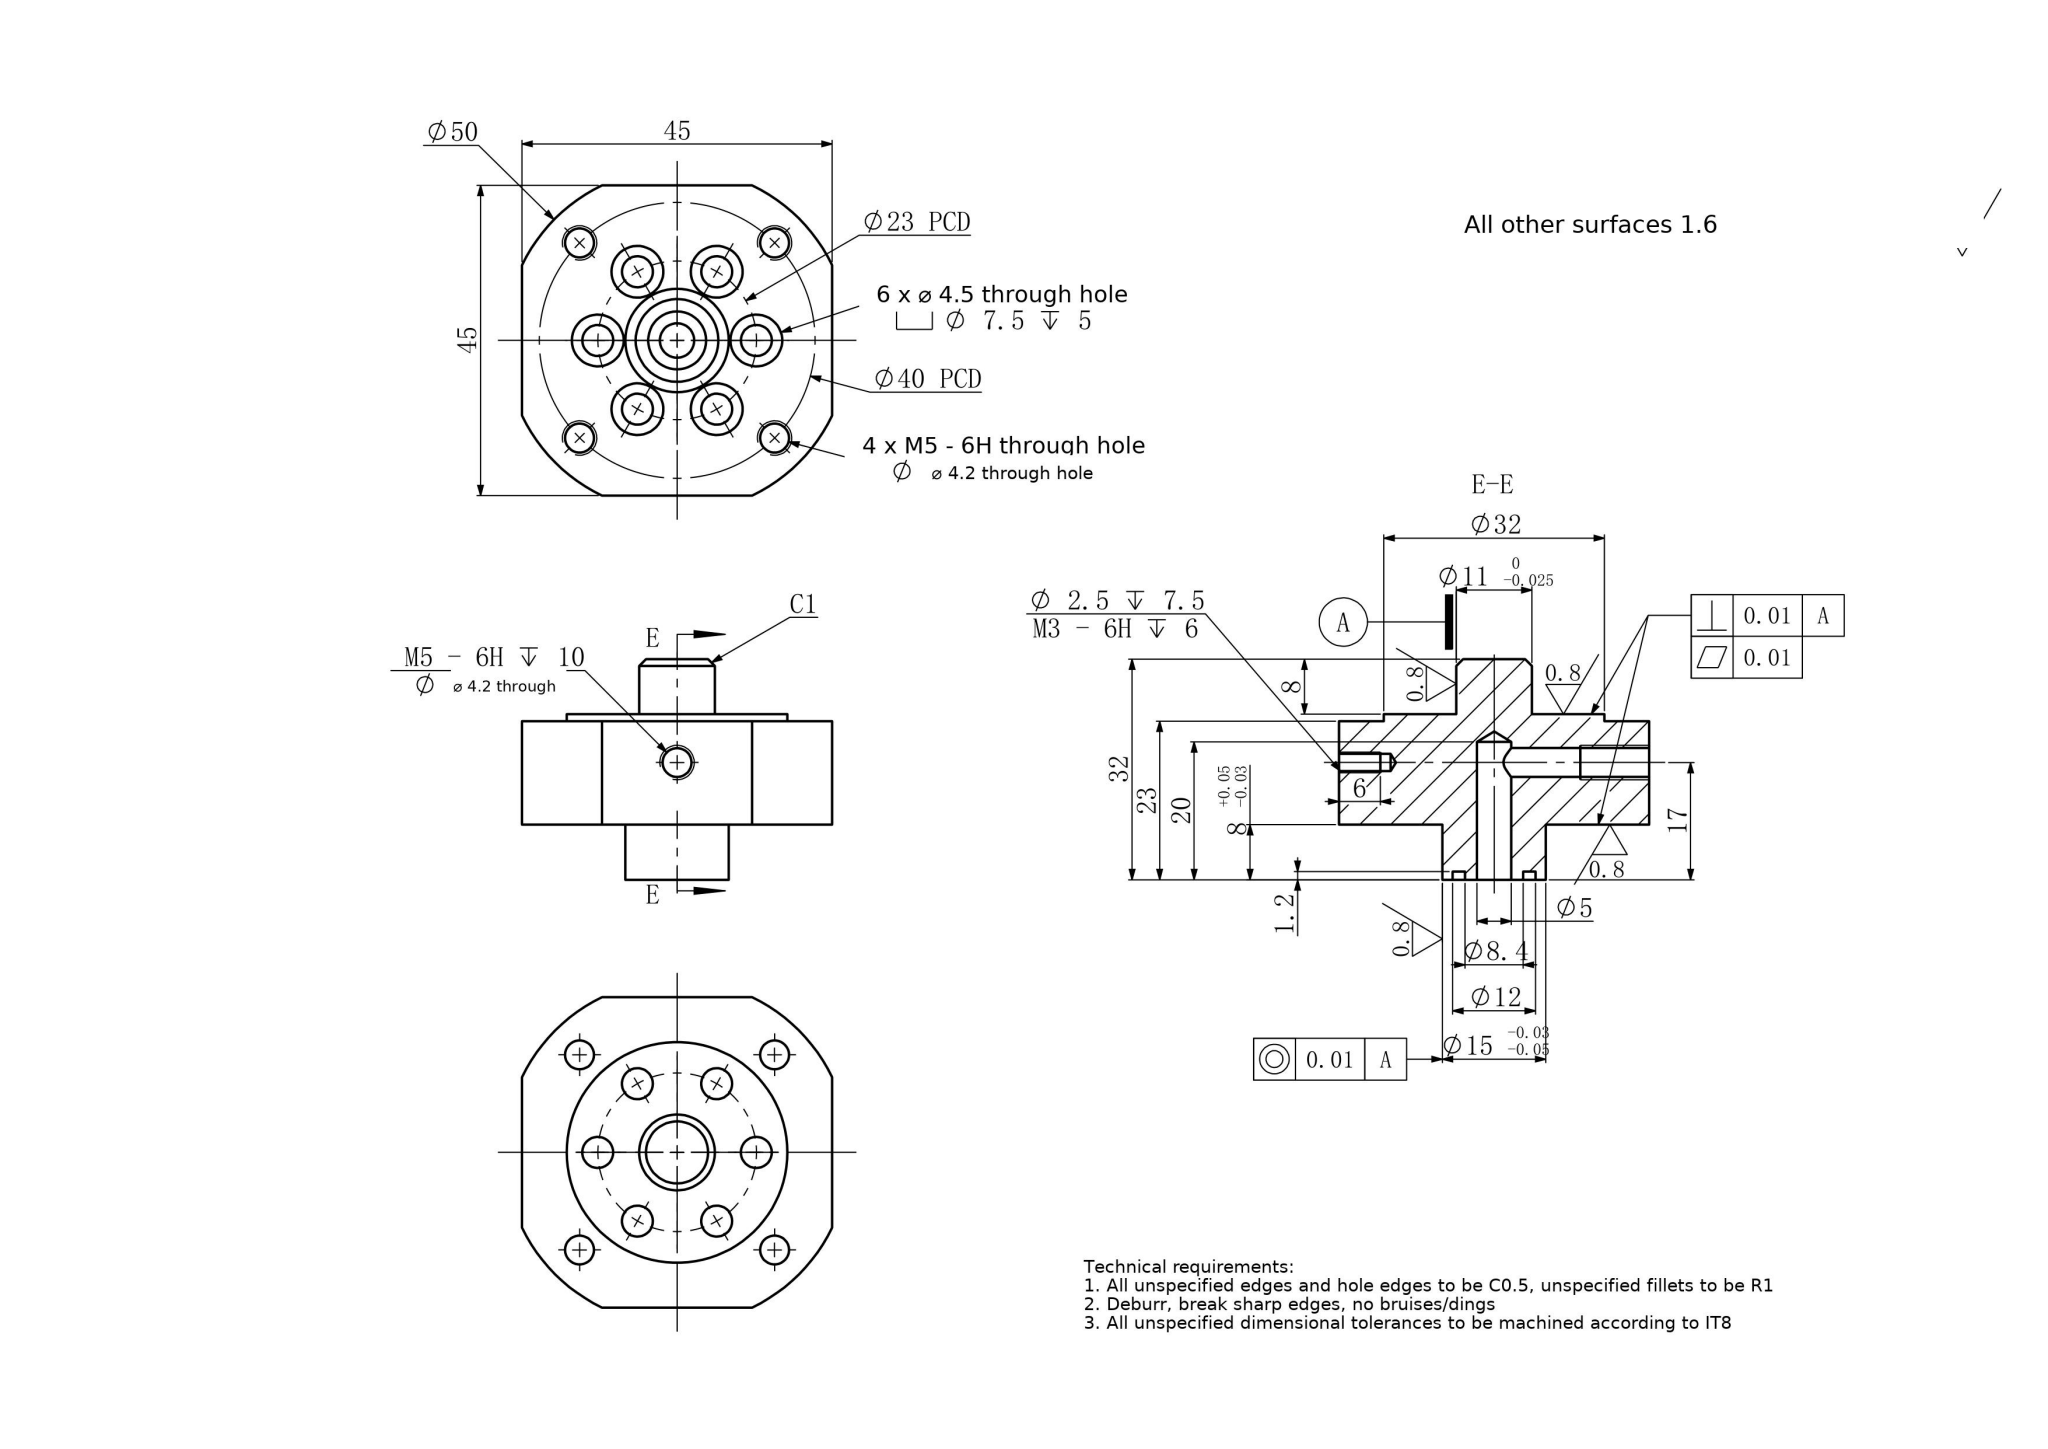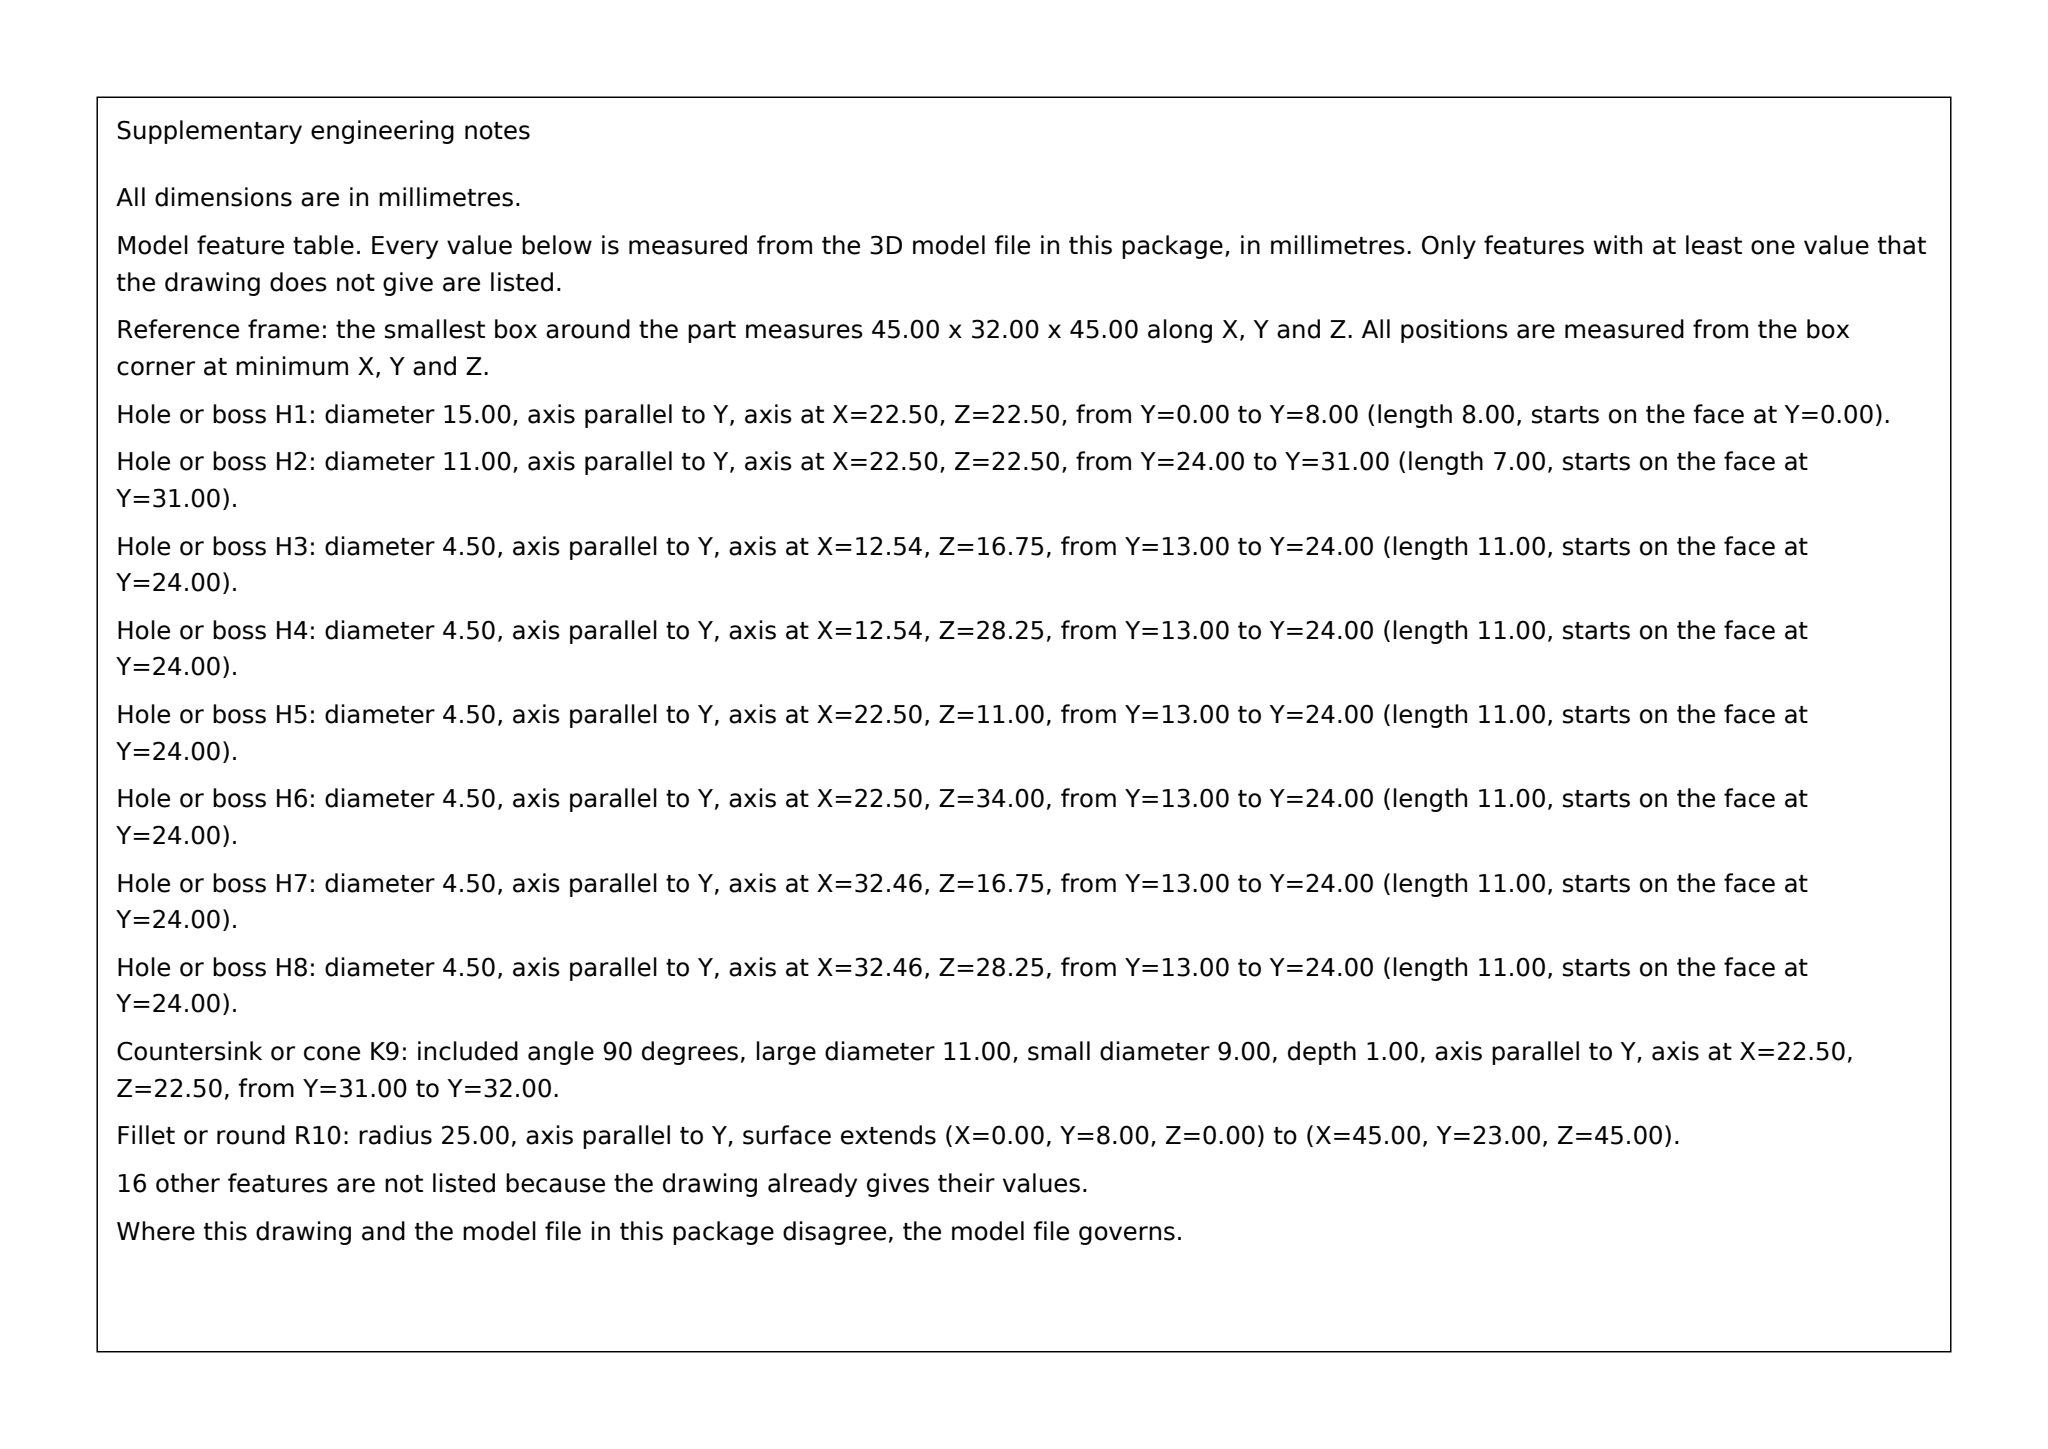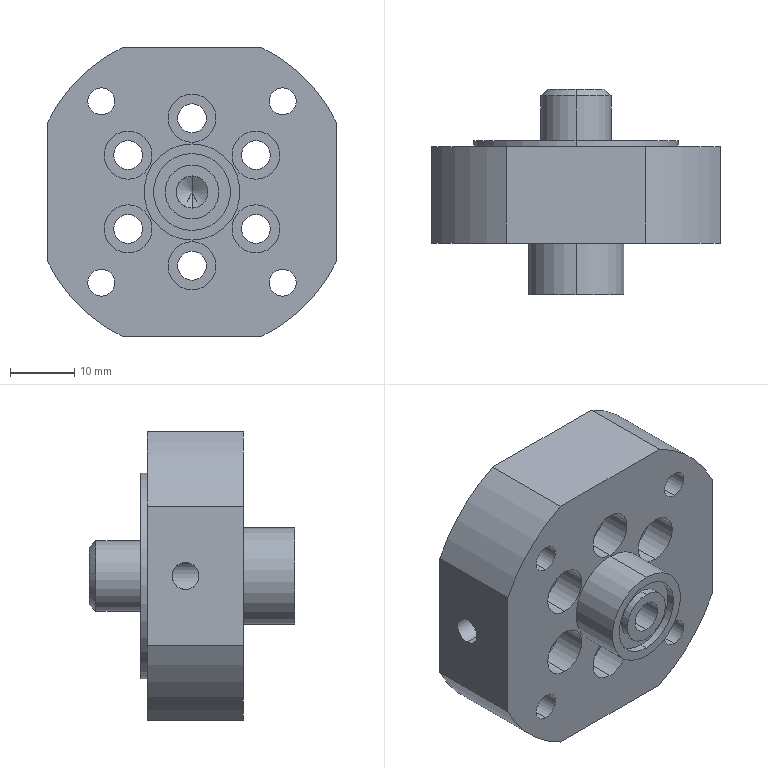Part | SolidWorks | mm | 1 solid | 75 faces | box 45 x 32 x 45 mm | volume 26216 mm3 | cylinder 52 | plane 17 | cone 6 | commonest cylinder face diameters 7.5 x12 4.5 x12 4.2 x10 50 x4 8.4 x2 12 x2 2.5 x2 5 x2